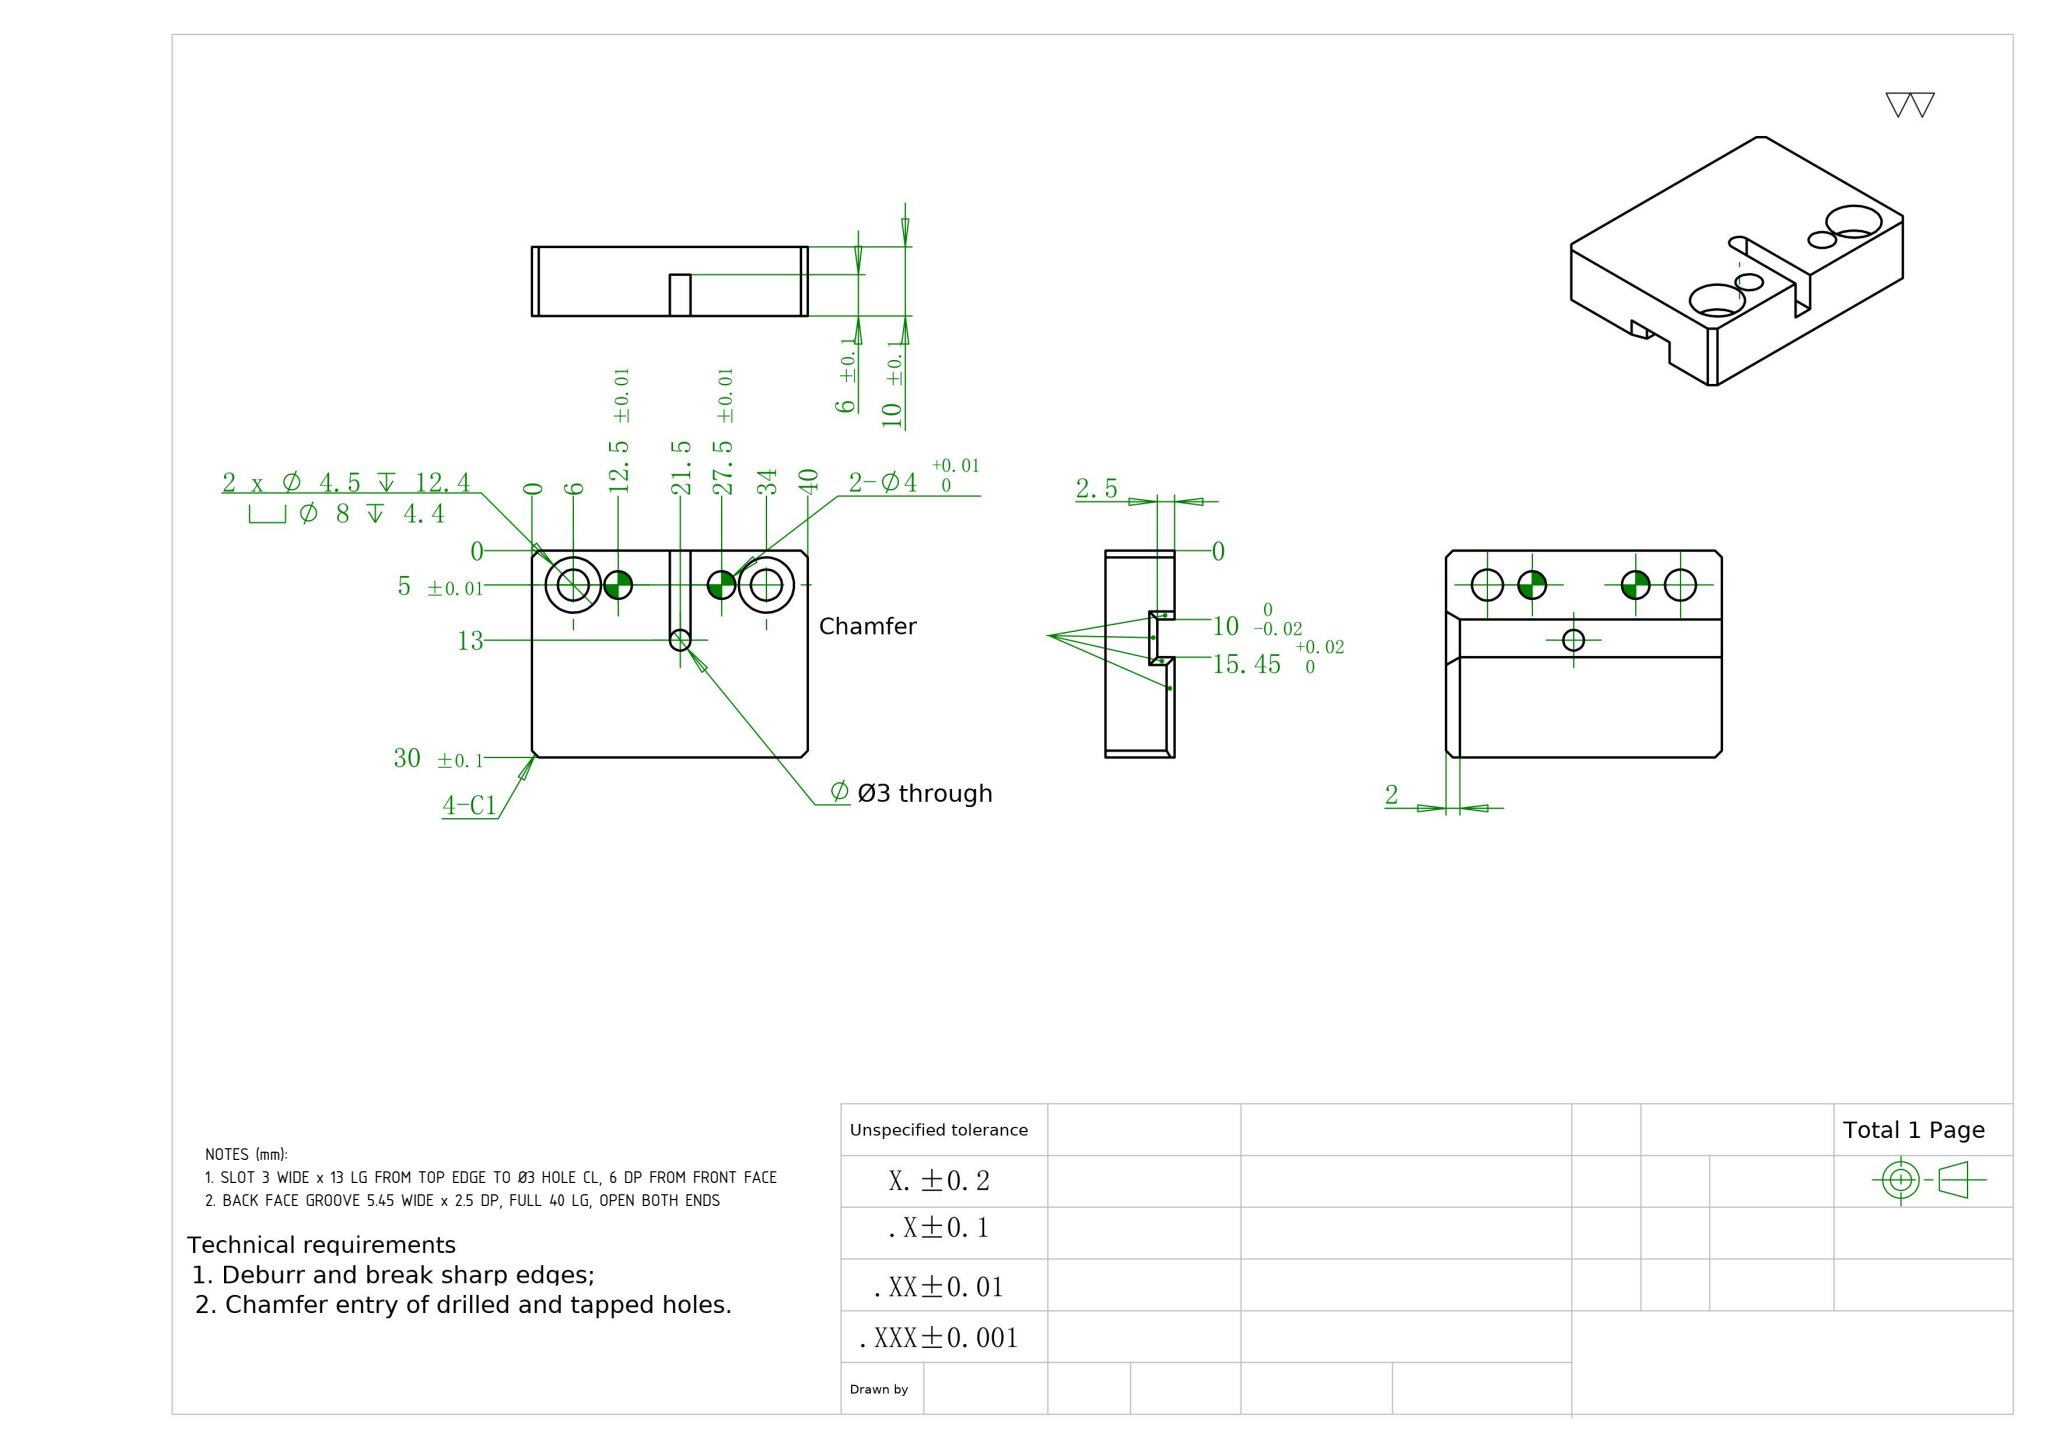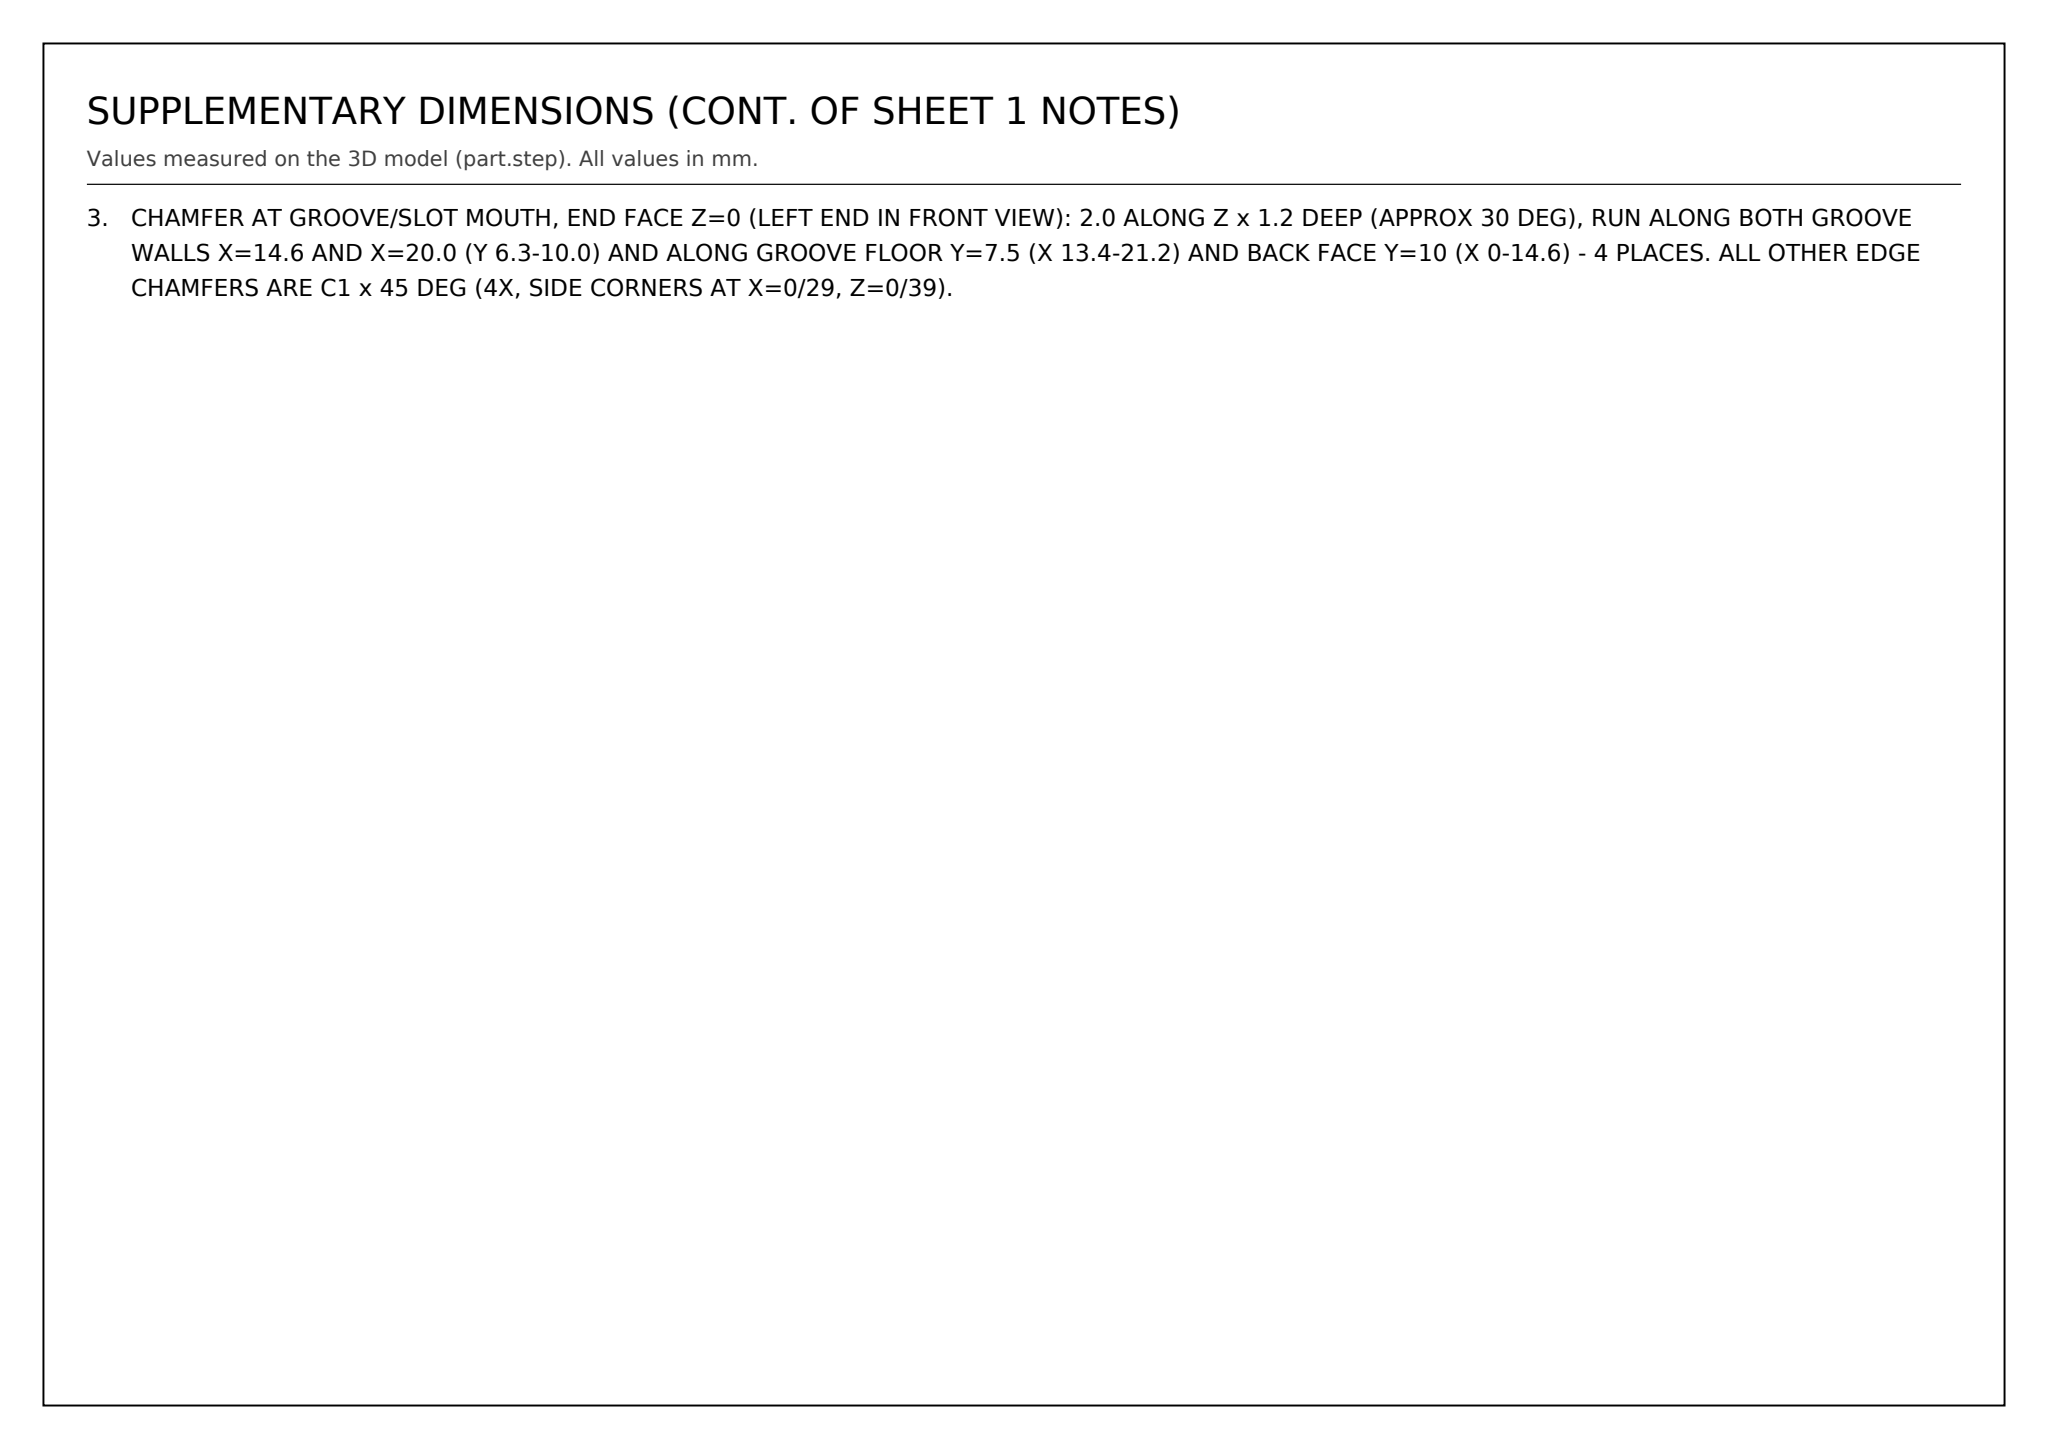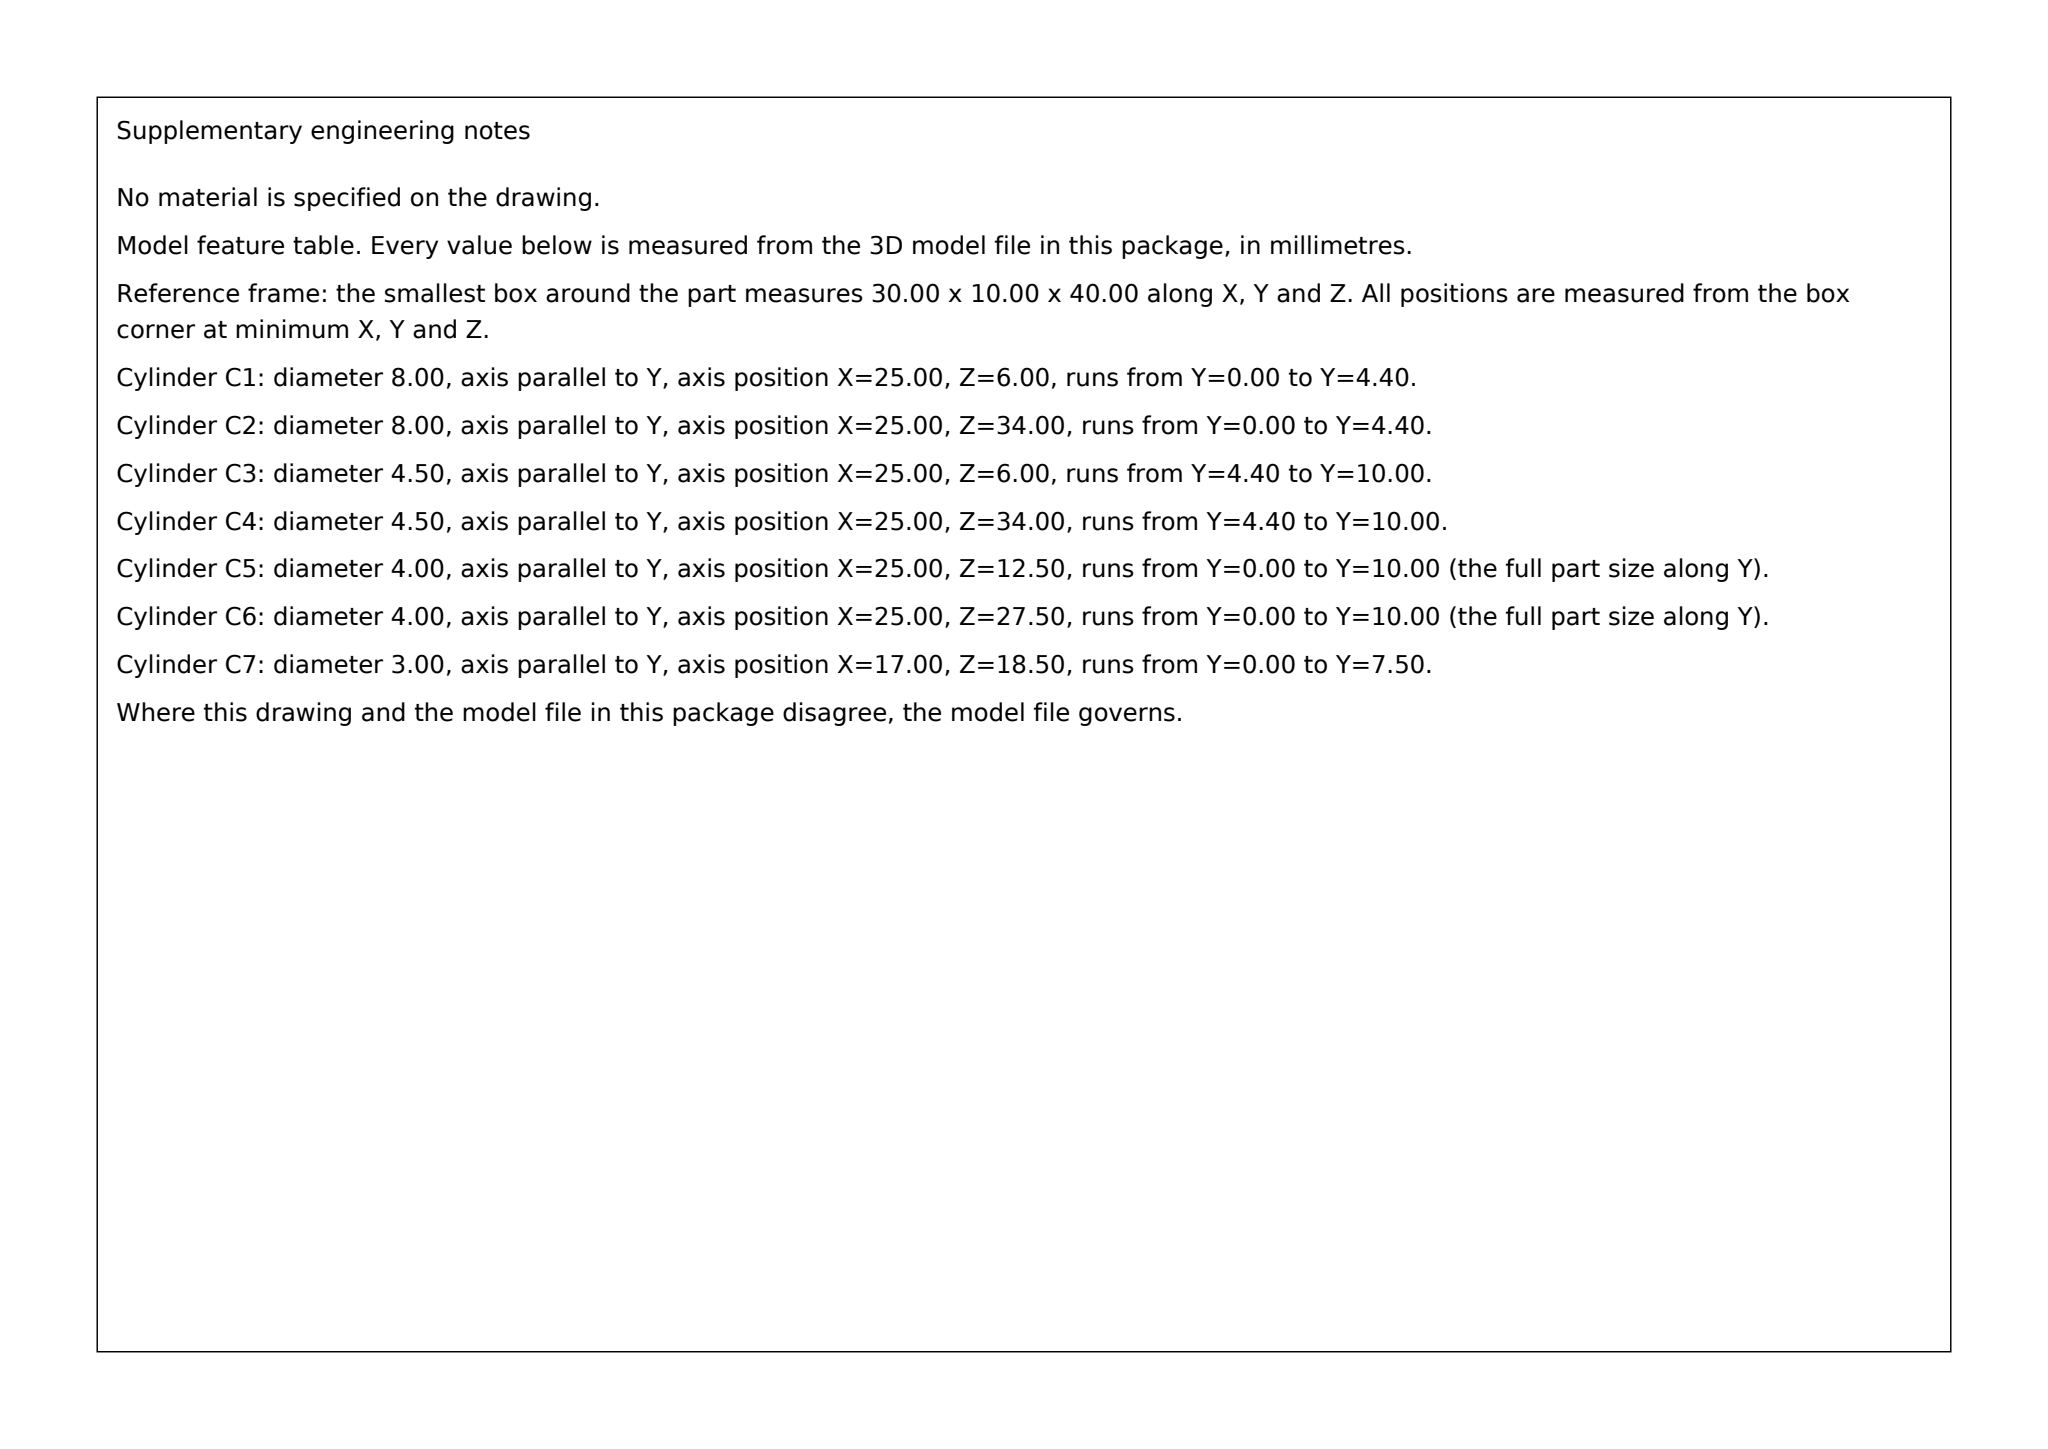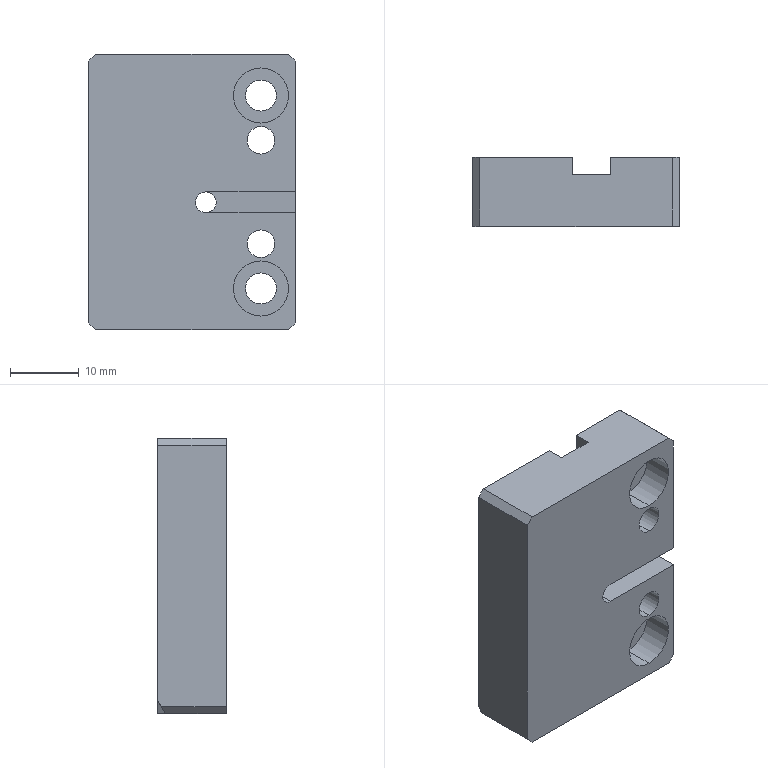Part | SolidWorks | mm | 1 solid | 37 faces | box 30 x 10 x 40 mm | volume 10268 mm3 | plane 23 | cylinder 14 | commonest cylinder face diameters 4 x4 8 x4 4.5 x4 3 x2
Drawing notes:
SLOT 3 WIDE x 13 LG FROM TOP EDGE TO Ø3 HOLE CL, 6 DP FROM FRONT FACE | from the solid: z-planes 17.0/20.0 = 3 wide, CL 18.5 (21.5 from datum); slot runs x=30 to Ø3 axis x=17 = 13 LG; y-plane 6.0 = slot floor 6 from front face y=0
BACK FACE GROOVE 5.45 WIDE x 2.5 DP, FULL 40 LG, OPEN BOTH ENDS | from the solid: x-planes 14.55/20.0 = 5.45 wide (10 to 15.45 from top edge x=30); y-planes 7.5 floor vs 10.0 back face = 2.5 DP; no z bounds, spans z 0-40
CHAMFER AT GROOVE/SLOT MOUTH, END FACE Z=0 (LEFT END IN FRONT VIEW): 2.0 ALONG Z x 1.2 DEEP (APPROX 30 DEG), RUN ALONG BOTH GROOVE WALLS X=14.6 AND X=20.0 (Y 6.3-10.0) AND ALONG GROOVE FLOOR Y=7.5 (X 13.4-21.2) AND BACK FACE Y=10 (X 0-14.6) - 4 PLACES. ALL OTHER EDGE CHAMFERS ARE C1 x 45 DEG (4X, SIDE CORNERS AT X=0/29, Z=0/39). | from the solid: inclined_planes: angle_to_xyz_axes [30,90,60] bbox_from [13.4,6.3,0] size [1.2,3.7,2.0]; [30,90,60] bbox_from [20.0,6.3,0] size [1.2,3.7,2.0]; [90,30,60] bbox_from [0,8.8,0] size [14.6,1.2,2.0]; [90,30,60] bbox_from [13.4,6.3,0] size [7.8,1.2,2.0]; plus 45 deg planes size [1.0,*,1.0] at x=0/29, z=0/39
build123d program:
from build123d import *
from OCP.BRepFilletAPI import BRepFilletAPI_MakeChamfer

# Parameters (mm, degrees)
BOSS_EXTRUDE1_DEPTH                             = 40
M4_HEX_SOCKET_HEAD_CAP_SCREW_CBORE1_D           = 4.5
M4_HEX_SOCKET_HEAD_CAP_SCREW_CBORE1_DEPTH       = 12.4
M4_HEX_SOCKET_HEAD_CAP_SCREW_CBORE1_CBORE_D     = 8
M4_HEX_SOCKET_HEAD_CAP_SCREW_CBORE1_CBORE_DEPTH = 4.4
M4_HEX_SOCKET_HEAD_CAP_SCREW_CBORE1_TIP         = 1.352
F_4_0_4_DIAMETER_HOLE1_D                        = 4
F_4_0_4_DIAMETER_HOLE1_DEPTH                    = 10
F_4_0_4_DIAMETER_HOLE1_TIP                      = 1.202
F_2_0_2_DIAMETER_HOLE1_D                        = 3
CHAMFER1_SIZE                                   = 2
CHAMFER1_SIZE2                                  = 1.155
CUT_EXTRUDE2_START                              = -6
CUT_EXTRUDE2_DEPTH                              = 6
CHAMFER2_SIZE                                   = 1


with BuildPart() as part:
    # Sketch1 → Boss-Extrude1 (new body)
    with BuildSketch(Plane.XY):
        Polygon((0, 0), (0, 10), (14.55, 10), (14.55, 7.5), (20, 7.5), (20, 10), (30, 10), (30, 0), align=None)
    extrude(amount=BOSS_EXTRUDE1_DEPTH)

    # M4 Hex Socket Head Cap Screw CBORE1
    with Locations(Plane(origin=(0, 0, 0), x_dir=(-1, 0, 0), z_dir=(0, -1, 0))):
        with Locations((-25, -34), (-25, -6)):
            CounterBoreHole(M4_HEX_SOCKET_HEAD_CAP_SCREW_CBORE1_D / 2, M4_HEX_SOCKET_HEAD_CAP_SCREW_CBORE1_CBORE_D / 2, M4_HEX_SOCKET_HEAD_CAP_SCREW_CBORE1_CBORE_DEPTH, depth=M4_HEX_SOCKET_HEAD_CAP_SCREW_CBORE1_DEPTH)
            with Locations((0, 0, -(M4_HEX_SOCKET_HEAD_CAP_SCREW_CBORE1_DEPTH + M4_HEX_SOCKET_HEAD_CAP_SCREW_CBORE1_TIP / 2))):  # 118° drill point
                Cone(0, M4_HEX_SOCKET_HEAD_CAP_SCREW_CBORE1_D / 2, M4_HEX_SOCKET_HEAD_CAP_SCREW_CBORE1_TIP, mode=Mode.SUBTRACT)

    # 4.0 _4_ Diameter Hole1
    with Locations(Plane(origin=(0, 0, 0), x_dir=(-1, 0, 0), z_dir=(0, -1, 0))):
        with Locations((-25, -27.5), (-25, -12.5)):
            Hole(F_4_0_4_DIAMETER_HOLE1_D / 2, depth=F_4_0_4_DIAMETER_HOLE1_DEPTH)
            with Locations((0, 0, -(F_4_0_4_DIAMETER_HOLE1_DEPTH + F_4_0_4_DIAMETER_HOLE1_TIP / 2))):  # 118° drill point
                Cone(0, F_4_0_4_DIAMETER_HOLE1_D / 2, F_4_0_4_DIAMETER_HOLE1_TIP, mode=Mode.SUBTRACT)

    # 2.0 _2_ Diameter Hole1 (through all)
    with Locations(Plane(origin=(0, 0, 0), x_dir=(-1, 0, 0), z_dir=(0, -1, 0))):
        with Locations((-17, -18.5)):
            Hole(F_2_0_2_DIAMETER_HOLE1_D / 2)

    # Chamfer1: one chamfer whose edges measure the first distance from different faces: ONE call of the kernel's chamfer builder (chamfer() names one face for all edges)
    chamfer1_edges_1 = [part.edges().sort_by_distance(p)[0] for p in [
        (14.55, 8.75, 0),
    ]]
    chamfer1_side_1 = [part.faces().sort_by_distance(p)[0] for p in [
        (14.55, 8.75, 20),
    ]]
    chamfer1_edges_2 = [part.edges().sort_by_distance(p)[0] for p in [
        (17.275, 7.5, 0),
    ]]
    chamfer1_side_2 = [part.faces().sort_by_distance(p)[0] for p in [
        (17.284, 7.5, 20.05),
    ]]
    chamfer1_edges_3 = [part.edges().sort_by_distance(p)[0] for p in [
        (20, 8.75, 0),
    ]]
    chamfer1_side_3 = [part.faces().sort_by_distance(p)[0] for p in [
        (20, 8.75, 20),
    ]]
    chamfer1_edges_4 = [part.edges().sort_by_distance(p)[0] for p in [
        (7.275, 10, 0),
    ]]
    chamfer1_side_4 = [part.faces().sort_by_distance(p)[0] for p in [
        (7.275, 10, 20),
    ]]
    chamfer1 = BRepFilletAPI_MakeChamfer(part.part.solid().wrapped)
    for e in chamfer1_edges_1:
        chamfer1.Add(CHAMFER1_SIZE, CHAMFER1_SIZE2, e.wrapped, chamfer1_side_1[0].wrapped)  # the first distance lies on this face
    for e in chamfer1_edges_2:
        chamfer1.Add(CHAMFER1_SIZE, CHAMFER1_SIZE2, e.wrapped, chamfer1_side_2[0].wrapped)  # the first distance lies on this face
    for e in chamfer1_edges_3:
        chamfer1.Add(CHAMFER1_SIZE, CHAMFER1_SIZE2, e.wrapped, chamfer1_side_3[0].wrapped)  # the first distance lies on this face
    for e in chamfer1_edges_4:
        chamfer1.Add(CHAMFER1_SIZE, CHAMFER1_SIZE2, e.wrapped, chamfer1_side_4[0].wrapped)  # the first distance lies on this face
    add(Compound.cast(chamfer1.Shape()), mode=Mode.REPLACE)

    # Sketch11 → Cut-Extrude2 (cut)
    with BuildSketch(Plane.XZ.offset(CUT_EXTRUDE2_START)):
        with BuildLine():
            Line((17, 20), (30, 20))
            ThreePointArc((30, 20), (31.5, 18.5), (30, 17))
            Line((30, 17), (17, 17))
            ThreePointArc((17, 17), (15.5, 18.5), (17, 20))
        make_face()
    extrude(amount=CUT_EXTRUDE2_DEPTH, mode=Mode.SUBTRACT)

    # Chamfer2
    chamfer2_edges = [part.edges().sort_by_distance(p)[0] for p in [
        (30, 5, 0),
        (0, 5, 40),
        (0, 4.423, 0),
        (30, 5, 40),
    ]]
    chamfer(chamfer2_edges, length=CHAMFER2_SIZE)


solid = part.part